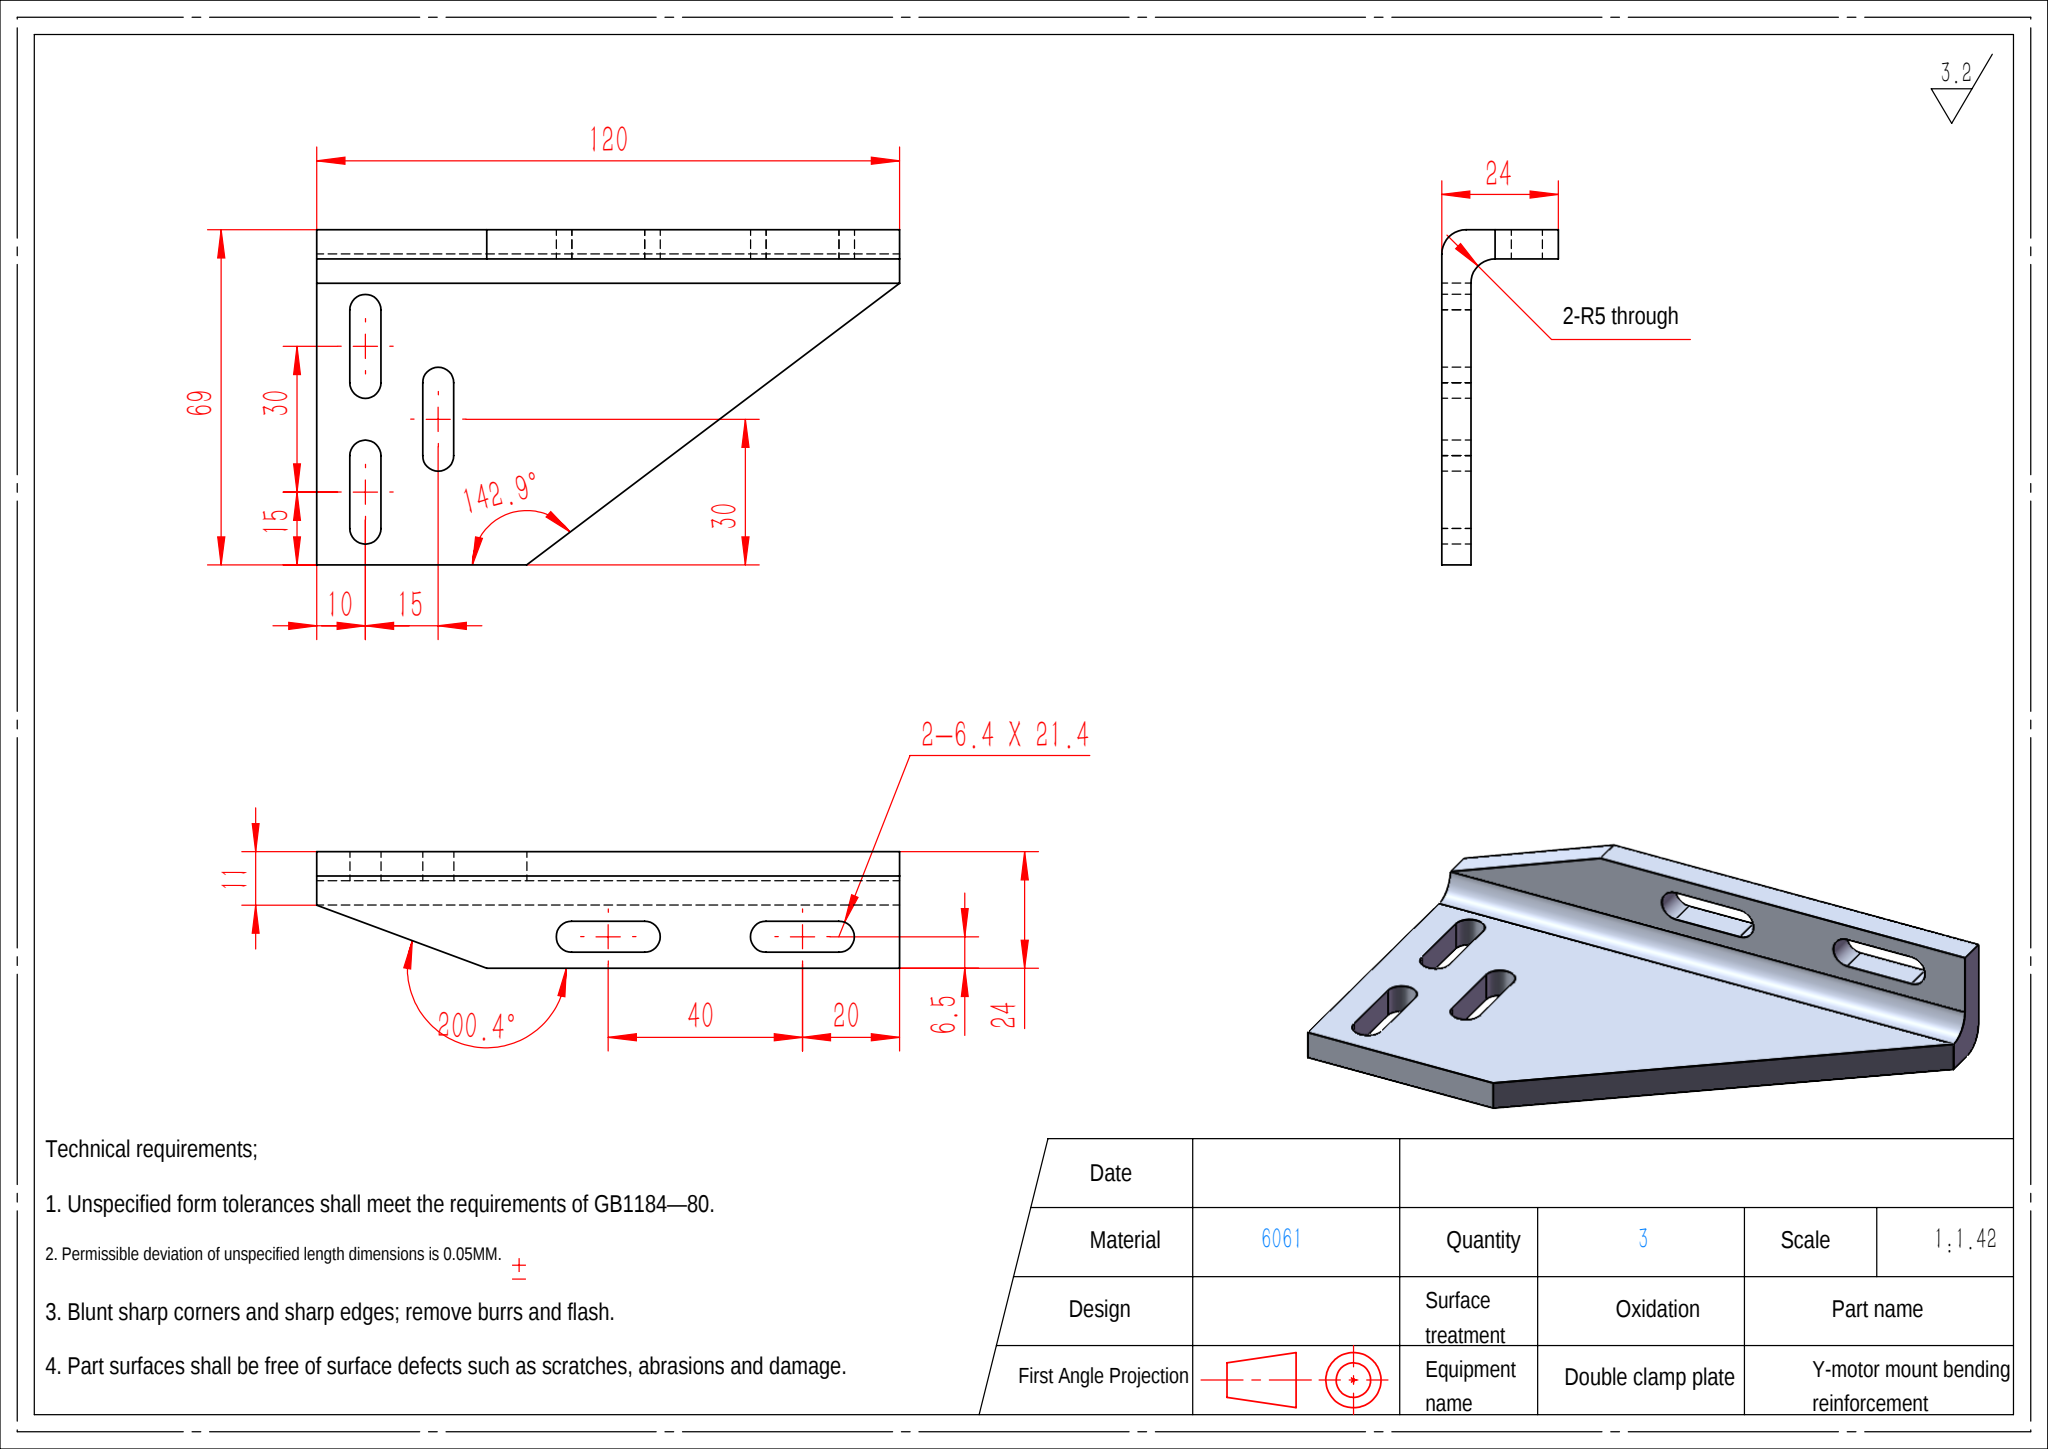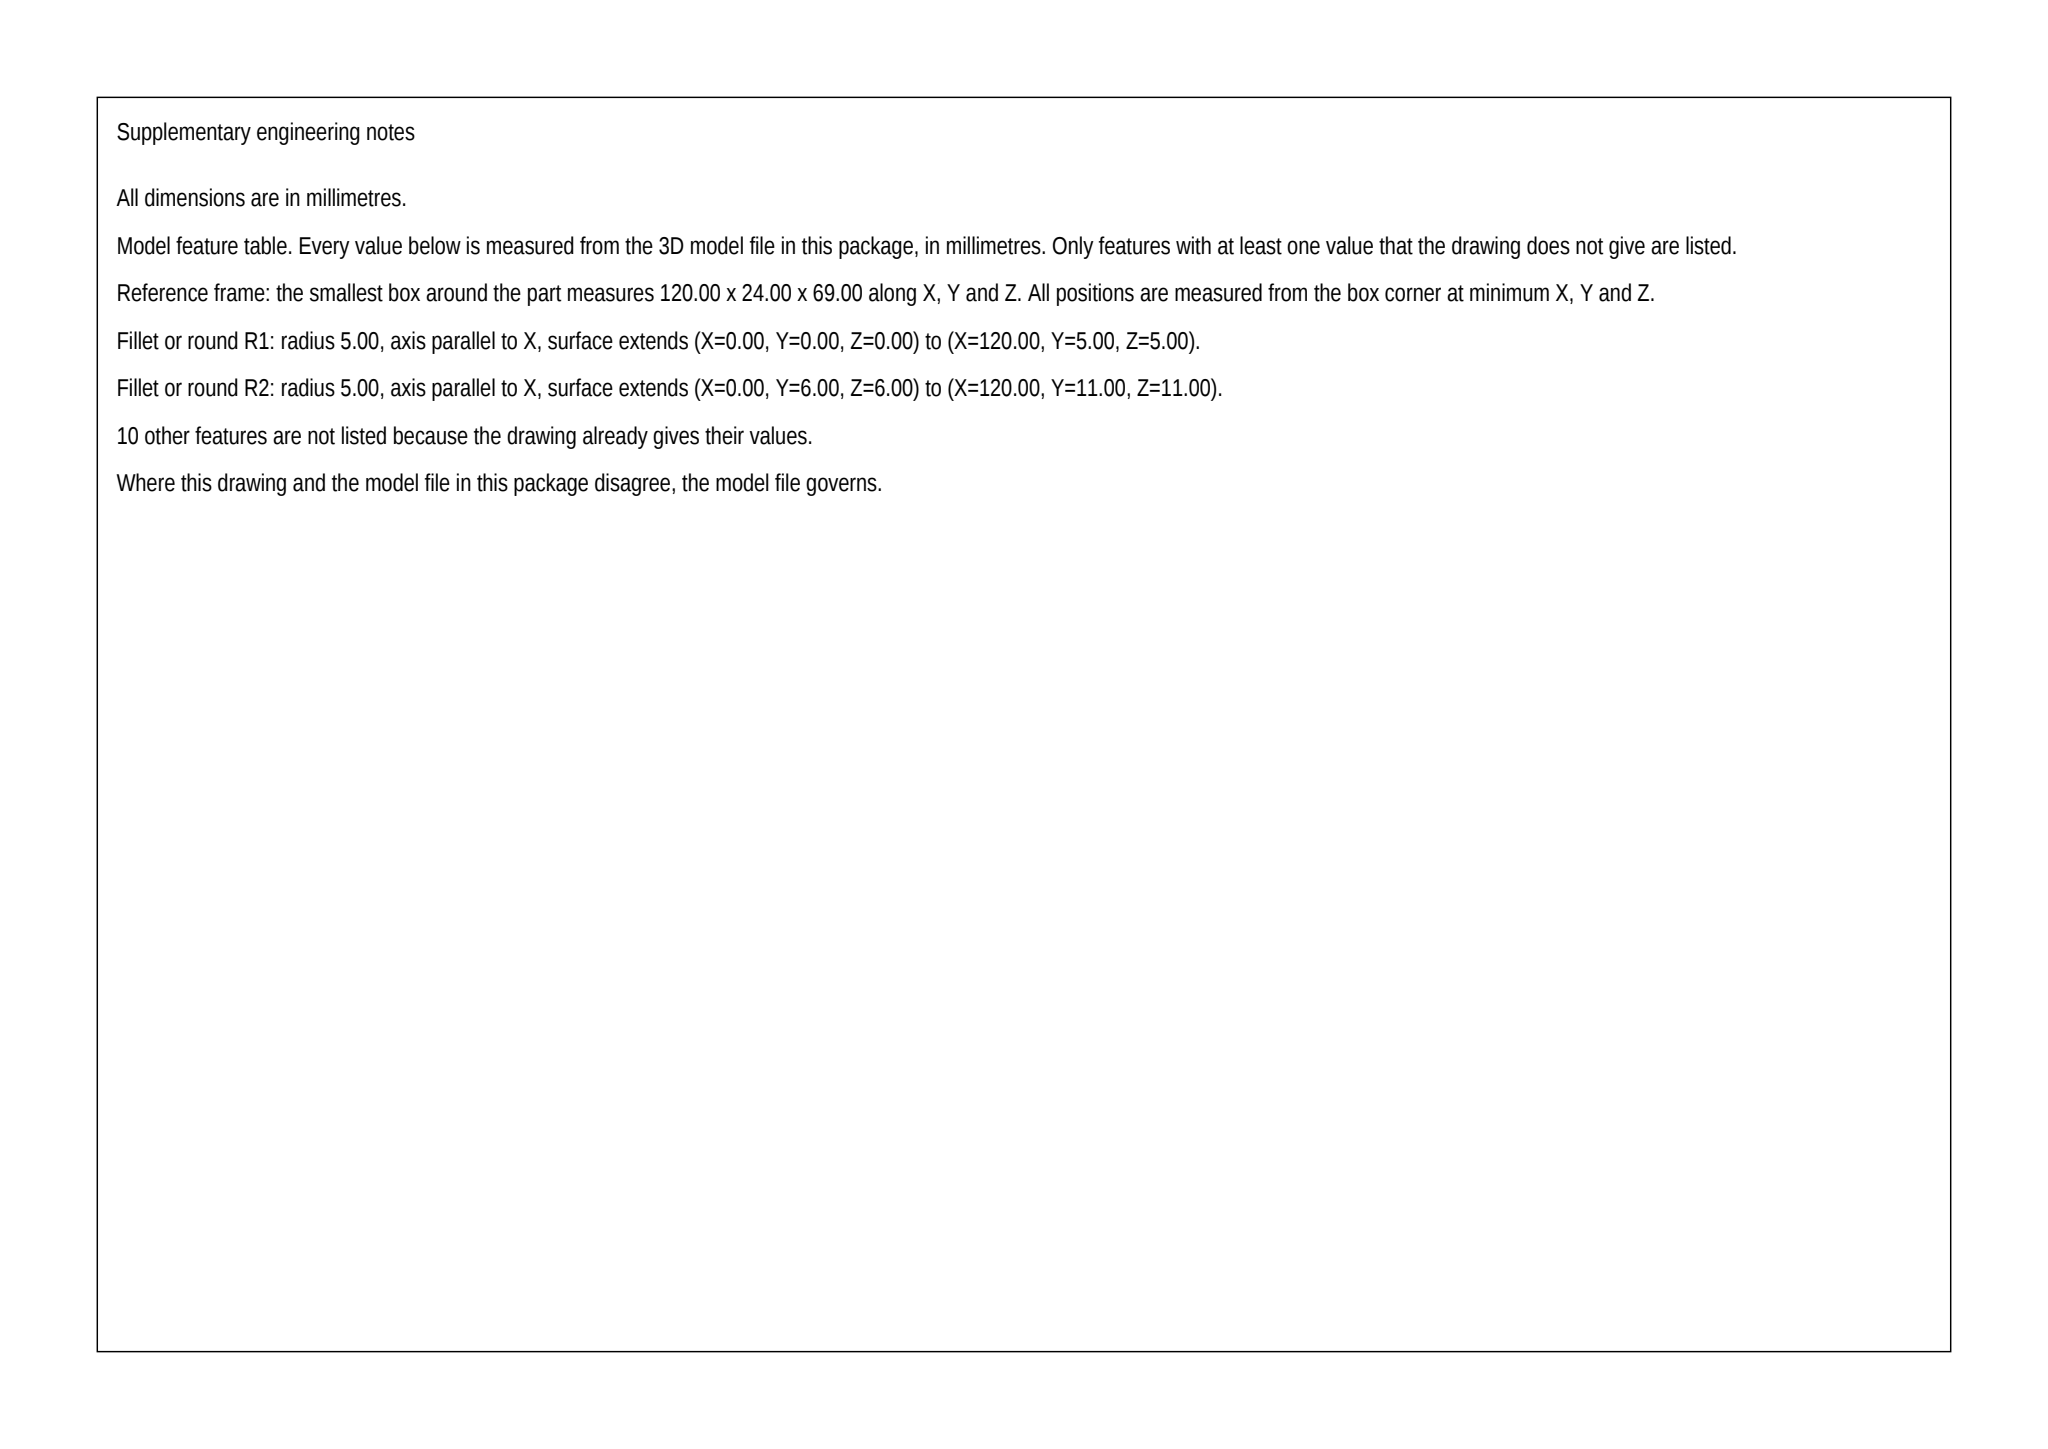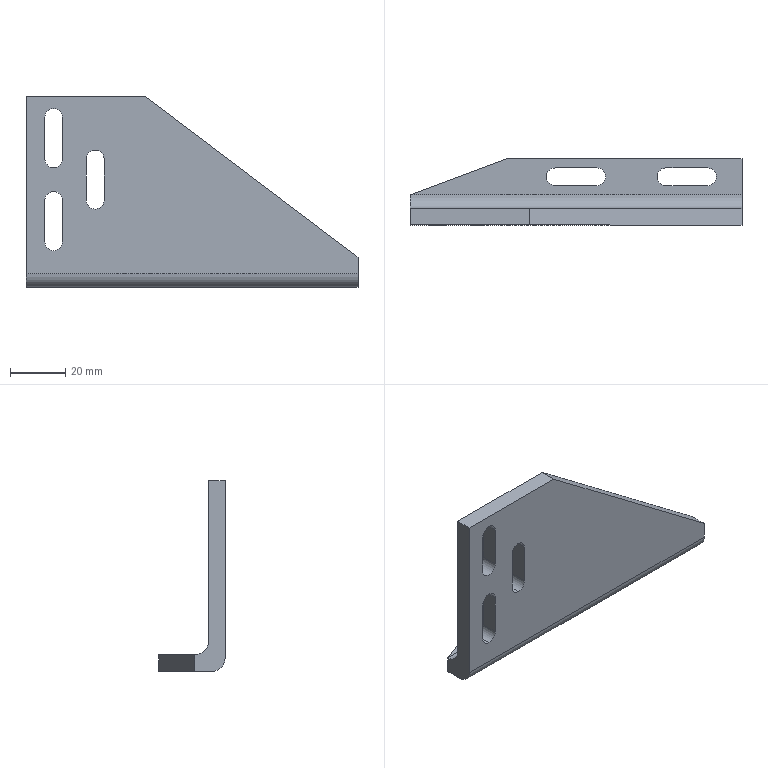Part | SolidWorks | mm | material 6061 | 1 solid | 37 faces | box 120 x 24 x 69 mm | volume 44073 mm3 | plane 20 | cylinder 17 | commonest cylinder face diameters 6.4 x15 10 x2